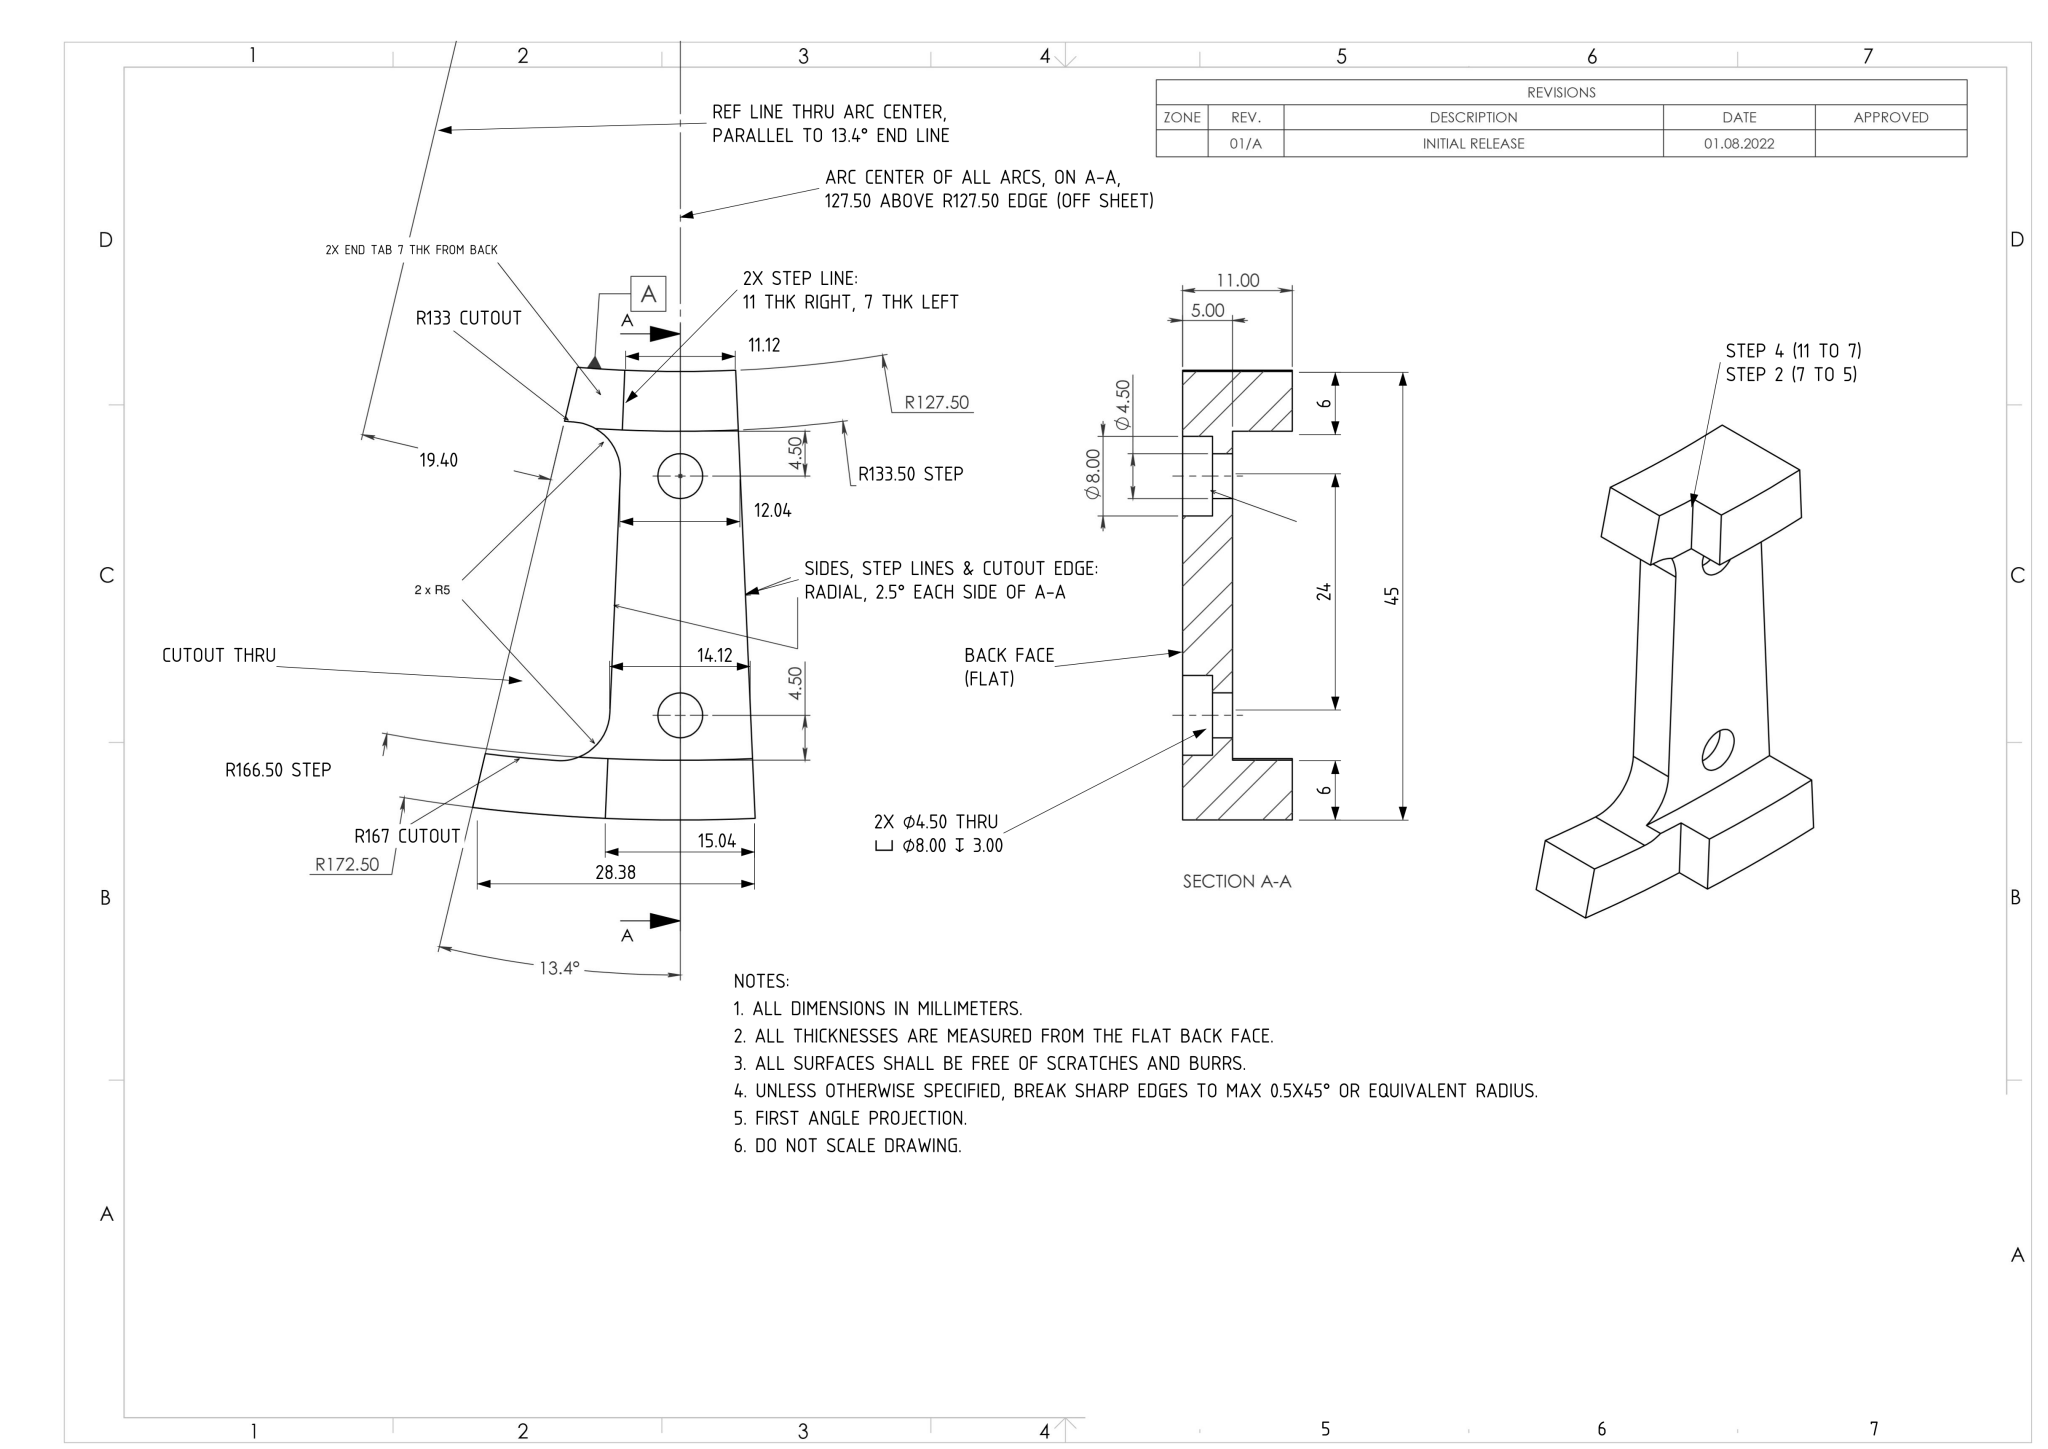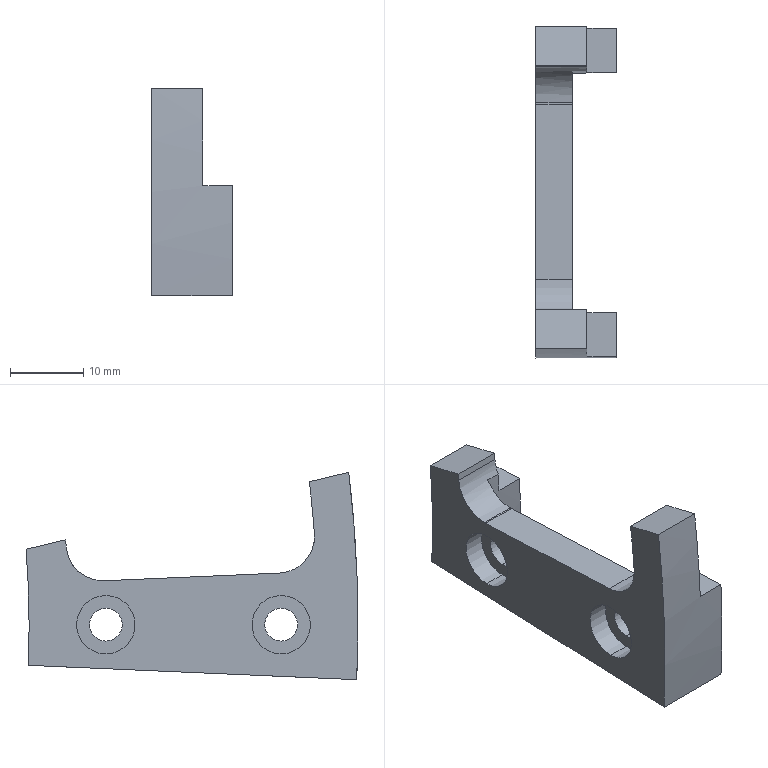Part | NX | mm | 1 solid | 31 faces | box 11 x 45.42 x 28.38 mm | volume 4282 mm3 | cylinder 17 | plane 14 | commonest cylinder face diameters 8 x4 4.5 x4 10 x3 345 x1 255 x1 267 x1 333 x1 266 x1
STEP:
#1=CARTESIAN_POINT('',(-7.131,-137.778,6.016));
#2=VERTEX_POINT('',#1);
#3=CARTESIAN_POINT('',(-7.131,-137.56,6.011));
#4=VERTEX_POINT('',#3);
#5=CARTESIAN_POINT('',(-7.131,-137.56,11.011));
#6=DIRECTION('',(1.,0.,0.));
#7=DIRECTION('',(0.,0.,-1.));
#8=AXIS2_PLACEMENT_3D('',#5,#6,#7);
#9=CIRCLE('',#8,5.);
#10=EDGE_CURVE('',#2,#4,#9,.T.);
#11=ORIENTED_EDGE('',*,*,#10,.T.);
#12=CARTESIAN_POINT('',(-12.131,-137.56,6.011));
#13=VERTEX_POINT('',#12);
#14=CARTESIAN_POINT('',(-5.131,-137.56,6.011));
#15=DIRECTION('',(-1.,0.,0.));
#16=VECTOR('',#15,1000.);
#17=LINE('',#14,#16);
#18=EDGE_CURVE('',#4,#13,#17,.T.);
#19=ORIENTED_EDGE('',*,*,#18,.T.);
#20=CARTESIAN_POINT('',(-12.131,-137.778,6.016));
#21=VERTEX_POINT('',#20);
#22=CARTESIAN_POINT('',(-12.131,-137.56,11.011));
#23=DIRECTION('',(-1.,0.,0.));
#24=DIRECTION('',(0.,0.,1.));
#25=AXIS2_PLACEMENT_3D('',#22,#23,#24);
#26=CIRCLE('',#25,5.);
#27=EDGE_CURVE('',#13,#21,#26,.T.);
#28=ORIENTED_EDGE('',*,*,#27,.T.);
#29=CARTESIAN_POINT('',(-5.131,-137.778,6.016));
#30=DIRECTION('',(1.,0.,0.));
#31=VECTOR('',#30,1000.);
#32=LINE('',#29,#31);
#33=EDGE_CURVE('',#21,#2,#32,.T.);
#34=ORIENTED_EDGE('',*,*,#33,.T.);
#35=EDGE_LOOP('',(#11,#19,#28,#34));
#36=FACE_OUTER_BOUND('',#35,.T.);
#37=CARTESIAN_POINT('',(-5.131,-137.56,11.011));
#38=DIRECTION('',(-1.,0.,0.));
#39=DIRECTION('',(0.,0.,-1.));
#40=AXIS2_PLACEMENT_3D('',#37,#38,#39);
#41=CYLINDRICAL_SURFACE('',#40,5.);
#42=ADVANCED_FACE('',(#36),#41,.F.);
#43=CARTESIAN_POINT('',(-9.131,-138.,-4.));
#44=VERTEX_POINT('',#43);
#45=CARTESIAN_POINT('',(-9.131,-138.,4.));
#46=VERTEX_POINT('',#45);
#47=CARTESIAN_POINT('',(-9.131,-138.,0.));
#48=DIRECTION('',(1.,0.,0.));
#49=DIRECTION('',(0.,0.,-1.));
#50=AXIS2_PLACEMENT_3D('',#47,#48,#49);
#51=CIRCLE('',#50,4.);
#52=EDGE_CURVE('',#44,#46,#51,.T.);
#53=ORIENTED_EDGE('',*,*,#52,.T.);
#54=CARTESIAN_POINT('',(-12.131,-138.,4.));
#55=VERTEX_POINT('',#54);
#56=CARTESIAN_POINT('',(-12.131,-138.,4.));
#57=DIRECTION('',(-1.,0.,0.));
#58=VECTOR('',#57,1000.);
#59=LINE('',#56,#58);
#60=EDGE_CURVE('',#46,#55,#59,.T.);
#61=ORIENTED_EDGE('',*,*,#60,.T.);
#62=CARTESIAN_POINT('',(-12.131,-138.,-4.));
#63=VERTEX_POINT('',#62);
#64=CARTESIAN_POINT('',(-12.131,-138.,0.));
#65=DIRECTION('',(1.,0.,0.));
#66=DIRECTION('',(0.,0.,-1.));
#67=AXIS2_PLACEMENT_3D('',#64,#65,#66);
#68=CIRCLE('',#67,4.);
#69=EDGE_CURVE('',#63,#55,#68,.T.);
#70=ORIENTED_EDGE('',*,*,#69,.F.);
#71=CARTESIAN_POINT('',(-12.131,-138.,-4.));
#72=DIRECTION('',(-1.,0.,0.));
#73=VECTOR('',#72,1000.);
#74=LINE('',#71,#73);
#75=EDGE_CURVE('',#44,#63,#74,.T.);
#76=ORIENTED_EDGE('',*,*,#75,.F.);
#77=EDGE_LOOP('',(#53,#61,#70,#76));
#78=FACE_OUTER_BOUND('',#77,.T.);
#79=CARTESIAN_POINT('',(-12.131,-138.,0.));
#80=DIRECTION('',(-1.,0.,0.));
#81=DIRECTION('',(0.,0.,-1.));
#82=AXIS2_PLACEMENT_3D('',#79,#80,#81);
#83=CYLINDRICAL_SURFACE('',#82,4.);
#84=ADVANCED_FACE('',(#78),#83,.F.);
#85=CARTESIAN_POINT('',(-7.131,-138.,-2.25));
#86=VERTEX_POINT('',#85);
#87=CARTESIAN_POINT('',(-7.131,-138.,2.25));
#88=VERTEX_POINT('',#87);
#89=CARTESIAN_POINT('',(-7.131,-138.,0.));
#90=DIRECTION('',(1.,0.,0.));
#91=DIRECTION('',(0.,0.,-1.));
#92=AXIS2_PLACEMENT_3D('',#89,#90,#91);
#93=CIRCLE('',#92,2.25);
#94=EDGE_CURVE('',#86,#88,#93,.T.);
#95=ORIENTED_EDGE('',*,*,#94,.T.);
#96=CARTESIAN_POINT('',(-9.131,-138.,2.25));
#97=VERTEX_POINT('',#96);
#98=CARTESIAN_POINT('',(-12.131,-138.,2.25));
#99=DIRECTION('',(-1.,0.,0.));
#100=VECTOR('',#99,1000.);
#101=LINE('',#98,#100);
#102=EDGE_CURVE('',#88,#97,#101,.T.);
#103=ORIENTED_EDGE('',*,*,#102,.T.);
#104=CARTESIAN_POINT('',(-9.131,-138.,-2.25));
#105=VERTEX_POINT('',#104);
#106=CARTESIAN_POINT('',(-9.131,-138.,0.));
#107=DIRECTION('',(1.,0.,0.));
#108=DIRECTION('',(0.,0.,-1.));
#109=AXIS2_PLACEMENT_3D('',#106,#107,#108);
#110=CIRCLE('',#109,2.25);
#111=EDGE_CURVE('',#105,#97,#110,.T.);
#112=ORIENTED_EDGE('',*,*,#111,.F.);
#113=CARTESIAN_POINT('',(-12.131,-138.,-2.25));
#114=DIRECTION('',(-1.,0.,0.));
#115=VECTOR('',#114,1000.);
#116=LINE('',#113,#115);
#117=EDGE_CURVE('',#86,#105,#116,.T.);
#118=ORIENTED_EDGE('',*,*,#117,.F.);
#119=EDGE_LOOP('',(#95,#103,#112,#118));
#120=FACE_OUTER_BOUND('',#119,.T.);
#121=CARTESIAN_POINT('',(-12.131,-138.,0.));
#122=DIRECTION('',(-1.,0.,0.));
#123=DIRECTION('',(0.,0.,-1.));
#124=AXIS2_PLACEMENT_3D('',#121,#122,#123);
#125=CYLINDRICAL_SURFACE('',#124,2.25);
#126=ADVANCED_FACE('',(#120),#125,.F.);
#127=CARTESIAN_POINT('',(-9.131,-162.,-4.));
#128=VERTEX_POINT('',#127);
#129=CARTESIAN_POINT('',(-9.131,-162.,4.));
#130=VERTEX_POINT('',#129);
#131=CARTESIAN_POINT('',(-9.131,-162.,0.));
#132=DIRECTION('',(1.,0.,0.));
#133=DIRECTION('',(0.,0.,-1.));
#134=AXIS2_PLACEMENT_3D('',#131,#132,#133);
#135=CIRCLE('',#134,4.);
#136=EDGE_CURVE('',#128,#130,#135,.T.);
#137=ORIENTED_EDGE('',*,*,#136,.T.);
#138=CARTESIAN_POINT('',(-12.131,-162.,4.));
#139=VERTEX_POINT('',#138);
#140=CARTESIAN_POINT('',(-12.131,-162.,4.));
#141=DIRECTION('',(-1.,0.,0.));
#142=VECTOR('',#141,1000.);
#143=LINE('',#140,#142);
#144=EDGE_CURVE('',#130,#139,#143,.T.);
#145=ORIENTED_EDGE('',*,*,#144,.T.);
#146=CARTESIAN_POINT('',(-12.131,-162.,-4.));
#147=VERTEX_POINT('',#146);
#148=CARTESIAN_POINT('',(-12.131,-162.,0.));
#149=DIRECTION('',(1.,0.,0.));
#150=DIRECTION('',(0.,0.,-1.));
#151=AXIS2_PLACEMENT_3D('',#148,#149,#150);
#152=CIRCLE('',#151,4.);
#153=EDGE_CURVE('',#147,#139,#152,.T.);
#154=ORIENTED_EDGE('',*,*,#153,.F.);
#155=CARTESIAN_POINT('',(-12.131,-162.,-4.));
#156=DIRECTION('',(-1.,0.,0.));
#157=VECTOR('',#156,1000.);
#158=LINE('',#155,#157);
#159=EDGE_CURVE('',#128,#147,#158,.T.);
#160=ORIENTED_EDGE('',*,*,#159,.F.);
#161=EDGE_LOOP('',(#137,#145,#154,#160));
#162=FACE_OUTER_BOUND('',#161,.T.);
#163=CARTESIAN_POINT('',(-12.131,-162.,0.));
#164=DIRECTION('',(-1.,0.,0.));
#165=DIRECTION('',(0.,0.,-1.));
#166=AXIS2_PLACEMENT_3D('',#163,#164,#165);
#167=CYLINDRICAL_SURFACE('',#166,4.);
#168=ADVANCED_FACE('',(#162),#167,.F.);
#169=CARTESIAN_POINT('',(-7.131,-162.,-2.25));
#170=VERTEX_POINT('',#169);
#171=CARTESIAN_POINT('',(-7.131,-162.,2.25));
#172=VERTEX_POINT('',#171);
#173=CARTESIAN_POINT('',(-7.131,-162.,0.));
#174=DIRECTION('',(1.,0.,0.));
#175=DIRECTION('',(0.,0.,-1.));
#176=AXIS2_PLACEMENT_3D('',#173,#174,#175);
#177=CIRCLE('',#176,2.25);
#178=EDGE_CURVE('',#170,#172,#177,.T.);
#179=ORIENTED_EDGE('',*,*,#178,.T.);
#180=CARTESIAN_POINT('',(-9.131,-162.,2.25));
#181=VERTEX_POINT('',#180);
#182=CARTESIAN_POINT('',(-12.131,-162.,2.25));
#183=DIRECTION('',(-1.,0.,0.));
#184=VECTOR('',#183,1000.);
#185=LINE('',#182,#184);
#186=EDGE_CURVE('',#172,#181,#185,.T.);
#187=ORIENTED_EDGE('',*,*,#186,.T.);
#188=CARTESIAN_POINT('',(-9.131,-162.,-2.25));
#189=VERTEX_POINT('',#188);
#190=CARTESIAN_POINT('',(-9.131,-162.,0.));
#191=DIRECTION('',(1.,0.,0.));
#192=DIRECTION('',(0.,0.,-1.));
#193=AXIS2_PLACEMENT_3D('',#190,#191,#192);
#194=CIRCLE('',#193,2.25);
#195=EDGE_CURVE('',#189,#181,#194,.T.);
#196=ORIENTED_EDGE('',*,*,#195,.F.);
#197=CARTESIAN_POINT('',(-12.131,-162.,-2.25));
#198=DIRECTION('',(-1.,0.,0.));
#199=VECTOR('',#198,1000.);
#200=LINE('',#197,#199);
#201=EDGE_CURVE('',#170,#189,#200,.T.);
#202=ORIENTED_EDGE('',*,*,#201,.F.);
#203=EDGE_LOOP('',(#179,#187,#196,#202));
#204=FACE_OUTER_BOUND('',#203,.T.);
#205=CARTESIAN_POINT('',(-12.131,-162.,0.));
#206=DIRECTION('',(-1.,0.,0.));
#207=DIRECTION('',(0.,0.,-1.));
#208=AXIS2_PLACEMENT_3D('',#205,#206,#207);
#209=CYLINDRICAL_SURFACE('',#208,2.25);
#210=ADVANCED_FACE('',(#204),#209,.F.);
#211=CARTESIAN_POINT('',(-7.131,-161.769,7.063));
#212=VERTEX_POINT('',#211);
#213=CARTESIAN_POINT('',(-7.131,-133.373,5.823));
#214=DIRECTION('',(-0.,0.999,-0.04362));
#215=VECTOR('',#214,1000.);
#216=LINE('',#213,#215);
#217=EDGE_CURVE('',#212,#2,#216,.T.);
#218=ORIENTED_EDGE('',*,*,#217,.T.);
#219=ORIENTED_EDGE('',*,*,#33,.F.);
#220=CARTESIAN_POINT('',(-12.131,-161.769,7.063));
#221=VERTEX_POINT('',#220);
#222=CARTESIAN_POINT('',(-12.131,-133.373,5.823));
#223=DIRECTION('',(0.,-0.999,0.04362));
#224=VECTOR('',#223,1000.);
#225=LINE('',#222,#224);
#226=EDGE_CURVE('',#21,#221,#225,.T.);
#227=ORIENTED_EDGE('',*,*,#226,.T.);
#228=CARTESIAN_POINT('',(-12.131,-161.769,7.063));
#229=DIRECTION('',(-1.,0.,0.));
#230=VECTOR('',#229,1000.);
#231=LINE('',#228,#230);
#232=EDGE_CURVE('',#212,#221,#231,.T.);
#233=ORIENTED_EDGE('',*,*,#232,.F.);
#234=EDGE_LOOP('',(#218,#219,#227,#233));
#235=FACE_OUTER_BOUND('',#234,.T.);
#236=CARTESIAN_POINT('',(0.,0.,0.));
#237=DIRECTION('',(0.,0.04362,0.999));
#238=DIRECTION('',(-1.,0.,0.));
#239=AXIS2_PLACEMENT_3D('',#236,#237,#238);
#240=PLANE('',#239);
#241=ADVANCED_FACE('',(#235),#240,.T.);
#242=CARTESIAN_POINT('',(-5.131,-172.336,7.524));
#243=VERTEX_POINT('',#242);
#244=CARTESIAN_POINT('',(-5.131,-166.342,7.263));
#245=VERTEX_POINT('',#244);
#246=CARTESIAN_POINT('',(-5.131,-166.841,7.284));
#247=DIRECTION('',(0.,0.999,-0.04362));
#248=VECTOR('',#247,1000.);
#249=LINE('',#246,#248);
#250=EDGE_CURVE('',#243,#245,#249,.T.);
#251=ORIENTED_EDGE('',*,*,#250,.F.);
#252=CARTESIAN_POINT('',(-1.131,-172.336,7.524));
#253=VERTEX_POINT('',#252);
#254=CARTESIAN_POINT('',(-12.131,-172.336,7.524));
#255=DIRECTION('',(1.,0.,0.));
#256=VECTOR('',#255,1000.);
#257=LINE('',#254,#256);
#258=EDGE_CURVE('',#243,#253,#257,.T.);
#259=ORIENTED_EDGE('',*,*,#258,.T.);
#260=CARTESIAN_POINT('',(-1.131,-166.342,7.263));
#261=VERTEX_POINT('',#260);
#262=CARTESIAN_POINT('',(-1.131,0.,0.));
#263=DIRECTION('',(0.,0.999,-0.04362));
#264=VECTOR('',#263,1000.);
#265=LINE('',#262,#264);
#266=EDGE_CURVE('',#253,#261,#265,.T.);
#267=ORIENTED_EDGE('',*,*,#266,.T.);
#268=CARTESIAN_POINT('',(-1.131,-166.342,7.263));
#269=DIRECTION('',(-1.,0.,0.));
#270=VECTOR('',#269,1000.);
#271=LINE('',#268,#270);
#272=EDGE_CURVE('',#261,#245,#271,.T.);
#273=ORIENTED_EDGE('',*,*,#272,.T.);
#274=EDGE_LOOP('',(#251,#259,#267,#273));
#275=FACE_OUTER_BOUND('',#274,.T.);
#276=CARTESIAN_POINT('',(0.,0.,0.));
#277=DIRECTION('',(0.,0.04362,0.999));
#278=DIRECTION('',(-1.,0.,0.));
#279=AXIS2_PLACEMENT_3D('',#276,#277,#278);
#280=PLANE('',#279);
#281=ADVANCED_FACE('',(#275),#280,.T.);
#282=CARTESIAN_POINT('',(-12.131,-127.379,-5.561));
#283=VERTEX_POINT('',#282);
#284=CARTESIAN_POINT('',(-12.131,-127.081,10.332));
#285=VERTEX_POINT('',#284);
#286=CARTESIAN_POINT('',(-12.131,0.,0.));
#287=DIRECTION('',(-1.,0.,0.));
#288=DIRECTION('',(0.,0.,1.));
#289=AXIS2_PLACEMENT_3D('',#286,#287,#288);
#290=CIRCLE('',#289,127.5);
#291=EDGE_CURVE('',#283,#285,#290,.T.);
#292=ORIENTED_EDGE('',*,*,#291,.F.);
#293=CARTESIAN_POINT('',(-12.131,-172.336,-7.524));
#294=VERTEX_POINT('',#293);
#295=CARTESIAN_POINT('',(-12.131,-133.373,-5.823));
#296=DIRECTION('',(0.,-0.999,-0.04362));
#297=VECTOR('',#296,1000.);
#298=LINE('',#295,#297);
#299=EDGE_CURVE('',#283,#294,#298,.T.);
#300=ORIENTED_EDGE('',*,*,#299,.T.);
#301=CARTESIAN_POINT('',(-12.131,-171.235,20.851));
#302=VERTEX_POINT('',#301);
#303=CARTESIAN_POINT('',(-12.131,0.,0.));
#304=DIRECTION('',(-1.,0.,0.));
#305=DIRECTION('',(0.,0.,1.));
#306=AXIS2_PLACEMENT_3D('',#303,#304,#305);
#307=CIRCLE('',#306,172.5);
#308=EDGE_CURVE('',#294,#302,#307,.T.);
#309=ORIENTED_EDGE('',*,*,#308,.T.);
#310=CARTESIAN_POINT('',(-12.131,-165.85,19.568));
#311=VERTEX_POINT('',#310);
#312=CARTESIAN_POINT('',(-12.131,-165.85,19.568));
#313=DIRECTION('',(0.,-0.9728,0.2317));
#314=VECTOR('',#313,1000.);
#315=LINE('',#312,#314);
#316=EDGE_CURVE('',#311,#302,#315,.T.);
#317=ORIENTED_EDGE('',*,*,#316,.F.);
#318=CARTESIAN_POINT('',(-12.131,-166.537,12.43));
#319=VERTEX_POINT('',#318);
#320=CARTESIAN_POINT('',(-12.131,0.,0.));
#321=DIRECTION('',(-1.,0.,0.));
#322=DIRECTION('',(0.,0.,-1.));
#323=AXIS2_PLACEMENT_3D('',#320,#321,#322);
#324=CIRCLE('',#323,167.);
#325=EDGE_CURVE('',#319,#311,#324,.T.);
#326=ORIENTED_EDGE('',*,*,#325,.F.);
#327=CARTESIAN_POINT('',(-12.131,-161.551,12.058));
#328=DIRECTION('',(-1.,0.,0.));
#329=DIRECTION('',(0.,0.,1.));
#330=AXIS2_PLACEMENT_3D('',#327,#328,#329);
#331=CIRCLE('',#330,5.);
#332=EDGE_CURVE('',#221,#319,#331,.T.);
#333=ORIENTED_EDGE('',*,*,#332,.F.);
#334=ORIENTED_EDGE('',*,*,#226,.F.);
#335=ORIENTED_EDGE('',*,*,#27,.F.);
#336=CARTESIAN_POINT('',(-12.131,-132.576,10.612));
#337=VERTEX_POINT('',#336);
#338=CARTESIAN_POINT('',(-12.131,-137.56,11.011));
#339=DIRECTION('',(-1.,0.,0.));
#340=DIRECTION('',(0.,0.,1.));
#341=AXIS2_PLACEMENT_3D('',#338,#339,#340);
#342=CIRCLE('',#341,5.);
#343=EDGE_CURVE('',#337,#13,#342,.T.);
#344=ORIENTED_EDGE('',*,*,#343,.F.);
#345=CARTESIAN_POINT('',(-12.131,-132.491,11.621));
#346=VERTEX_POINT('',#345);
#347=CARTESIAN_POINT('',(-12.131,0.,0.));
#348=DIRECTION('',(1.,0.,0.));
#349=DIRECTION('',(0.,0.,-1.));
#350=AXIS2_PLACEMENT_3D('',#347,#348,#349);
#351=CIRCLE('',#350,133.);
#352=EDGE_CURVE('',#346,#337,#351,.T.);
#353=ORIENTED_EDGE('',*,*,#352,.F.);
#354=CARTESIAN_POINT('',(-12.131,-127.081,10.332));
#355=DIRECTION('',(0.,-0.9728,0.2317));
#356=VECTOR('',#355,1000.);
#357=LINE('',#354,#356);
#358=EDGE_CURVE('',#285,#346,#357,.T.);
#359=ORIENTED_EDGE('',*,*,#358,.F.);
#360=EDGE_LOOP('',(#292,#300,#309,#317,#326,#333,#334,#335,#344,#353,#359));
#361=FACE_OUTER_BOUND('',#360,.T.);
#362=ORIENTED_EDGE('',*,*,#153,.T.);
#363=CARTESIAN_POINT('',(-12.131,-162.,0.));
#364=DIRECTION('',(1.,0.,0.));
#365=DIRECTION('',(0.,0.,-1.));
#366=AXIS2_PLACEMENT_3D('',#363,#364,#365);
#367=CIRCLE('',#366,4.);
#368=EDGE_CURVE('',#139,#147,#367,.T.);
#369=ORIENTED_EDGE('',*,*,#368,.T.);
#370=EDGE_LOOP('',(#362,#369));
#371=FACE_BOUND('',#370,.T.);
#372=ORIENTED_EDGE('',*,*,#69,.T.);
#373=CARTESIAN_POINT('',(-12.131,-138.,0.));
#374=DIRECTION('',(1.,0.,0.));
#375=DIRECTION('',(0.,0.,-1.));
#376=AXIS2_PLACEMENT_3D('',#373,#374,#375);
#377=CIRCLE('',#376,4.);
#378=EDGE_CURVE('',#55,#63,#377,.T.);
#379=ORIENTED_EDGE('',*,*,#378,.T.);
#380=EDGE_LOOP('',(#372,#379));
#381=FACE_BOUND('',#380,.T.);
#382=CARTESIAN_POINT('',(-12.131,-133.373,-5.823));
#383=DIRECTION('',(1.,0.,0.));
#384=DIRECTION('',(0.,0.,1.));
#385=AXIS2_PLACEMENT_3D('',#382,#383,#384);
#386=PLANE('',#385);
#387=ADVANCED_FACE('',(#361,#371,#381),#386,.F.);
#388=ORIENTED_EDGE('',*,*,#94,.F.);
#389=CARTESIAN_POINT('',(-7.131,-138.,0.));
#390=DIRECTION('',(1.,0.,0.));
#391=DIRECTION('',(0.,0.,-1.));
#392=AXIS2_PLACEMENT_3D('',#389,#390,#391);
#393=CIRCLE('',#392,2.25);
#394=EDGE_CURVE('',#88,#86,#393,.T.);
#395=ORIENTED_EDGE('',*,*,#394,.F.);
#396=EDGE_LOOP('',(#388,#395));
#397=FACE_BOUND('',#396,.T.);
#398=ORIENTED_EDGE('',*,*,#178,.F.);
#399=CARTESIAN_POINT('',(-7.131,-162.,0.));
#400=DIRECTION('',(1.,0.,0.));
#401=DIRECTION('',(0.,0.,-1.));
#402=AXIS2_PLACEMENT_3D('',#399,#400,#401);
#403=CIRCLE('',#402,2.25);
#404=EDGE_CURVE('',#172,#170,#403,.T.);
#405=ORIENTED_EDGE('',*,*,#404,.F.);
#406=EDGE_LOOP('',(#398,#405));
#407=FACE_BOUND('',#406,.T.);
#408=CARTESIAN_POINT('',(-7.131,-166.342,-7.263));
#409=VERTEX_POINT('',#408);
#410=CARTESIAN_POINT('',(-7.131,-133.373,-5.823));
#411=VERTEX_POINT('',#410);
#412=CARTESIAN_POINT('',(-7.131,-133.373,-5.823));
#413=DIRECTION('',(-0.,0.999,0.04362));
#414=VECTOR('',#413,1000.);
#415=LINE('',#412,#414);
#416=EDGE_CURVE('',#409,#411,#415,.T.);
#417=ORIENTED_EDGE('',*,*,#416,.T.);
#418=CARTESIAN_POINT('',(-7.131,-133.228,8.514));
#419=VERTEX_POINT('',#418);
#420=CARTESIAN_POINT('',(-7.131,0.,0.));
#421=DIRECTION('',(-1.,0.,0.));
#422=DIRECTION('',(0.,0.,1.));
#423=AXIS2_PLACEMENT_3D('',#420,#421,#422);
#424=CIRCLE('',#423,133.5);
#425=EDGE_CURVE('',#411,#419,#424,.T.);
#426=ORIENTED_EDGE('',*,*,#425,.T.);
#427=CARTESIAN_POINT('',(-7.131,-137.56,11.011));
#428=DIRECTION('',(1.,0.,0.));
#429=DIRECTION('',(0.,0.,-1.));
#430=AXIS2_PLACEMENT_3D('',#427,#428,#429);
#431=CIRCLE('',#430,5.);
#432=EDGE_CURVE('',#4,#419,#431,.T.);
#433=ORIENTED_EDGE('',*,*,#432,.F.);
#434=ORIENTED_EDGE('',*,*,#10,.F.);
#435=ORIENTED_EDGE('',*,*,#217,.F.);
#436=CARTESIAN_POINT('',(-7.131,-166.188,10.189));
#437=VERTEX_POINT('',#436);
#438=CARTESIAN_POINT('',(-7.131,-161.551,12.058));
#439=DIRECTION('',(1.,0.,0.));
#440=DIRECTION('',(0.,0.,-1.));
#441=AXIS2_PLACEMENT_3D('',#438,#439,#440);
#442=CIRCLE('',#441,5.);
#443=EDGE_CURVE('',#437,#212,#442,.T.);
#444=ORIENTED_EDGE('',*,*,#443,.F.);
#445=CARTESIAN_POINT('',(-7.131,0.,0.));
#446=DIRECTION('',(-1.,0.,0.));
#447=DIRECTION('',(0.,0.,1.));
#448=AXIS2_PLACEMENT_3D('',#445,#446,#447);
#449=CIRCLE('',#448,166.5);
#450=EDGE_CURVE('',#409,#437,#449,.T.);
#451=ORIENTED_EDGE('',*,*,#450,.F.);
#452=EDGE_LOOP('',(#417,#426,#433,#434,#435,#444,#451));
#453=FACE_OUTER_BOUND('',#452,.T.);
#454=CARTESIAN_POINT('',(-7.131,-133.373,-5.823));
#455=DIRECTION('',(-1.,0.,0.));
#456=DIRECTION('',(0.,0.,-1.));
#457=AXIS2_PLACEMENT_3D('',#454,#455,#456);
#458=PLANE('',#457);
#459=ADVANCED_FACE('',(#397,#407,#453),#458,.F.);
#460=ORIENTED_EDGE('',*,*,#308,.F.);
#461=CARTESIAN_POINT('',(-1.131,-172.336,-7.524));
#462=VERTEX_POINT('',#461);
#463=CARTESIAN_POINT('',(0.,-172.336,-7.524));
#464=DIRECTION('',(1.,0.,0.));
#465=VECTOR('',#464,1000.);
#466=LINE('',#463,#465);
#467=EDGE_CURVE('',#294,#462,#466,.T.);
#468=ORIENTED_EDGE('',*,*,#467,.T.);
#469=CARTESIAN_POINT('',(-1.131,0.,0.));
#470=DIRECTION('',(-1.,0.,0.));
#471=DIRECTION('',(0.,0.,1.));
#472=AXIS2_PLACEMENT_3D('',#469,#470,#471);
#473=CIRCLE('',#472,172.5);
#474=EDGE_CURVE('',#462,#253,#473,.T.);
#475=ORIENTED_EDGE('',*,*,#474,.T.);
#476=ORIENTED_EDGE('',*,*,#258,.F.);
#477=CARTESIAN_POINT('',(-5.131,-171.235,20.851));
#478=VERTEX_POINT('',#477);
#479=CARTESIAN_POINT('',(-5.131,0.,0.));
#480=DIRECTION('',(1.,0.,0.));
#481=DIRECTION('',(0.,0.,-1.));
#482=AXIS2_PLACEMENT_3D('',#479,#480,#481);
#483=CIRCLE('',#482,172.5);
#484=EDGE_CURVE('',#478,#243,#483,.T.);
#485=ORIENTED_EDGE('',*,*,#484,.F.);
#486=CARTESIAN_POINT('',(-5.131,-171.235,20.851));
#487=DIRECTION('',(-1.,0.,0.));
#488=VECTOR('',#487,1000.);
#489=LINE('',#486,#488);
#490=EDGE_CURVE('',#478,#302,#489,.T.);
#491=ORIENTED_EDGE('',*,*,#490,.T.);
#492=EDGE_LOOP('',(#460,#468,#475,#476,#485,#491));
#493=FACE_OUTER_BOUND('',#492,.T.);
#494=CARTESIAN_POINT('',(0.,0.,0.));
#495=DIRECTION('',(1.,0.,0.));
#496=DIRECTION('',(0.,0.,1.));
#497=AXIS2_PLACEMENT_3D('',#494,#495,#496);
#498=CYLINDRICAL_SURFACE('',#497,172.5);
#499=ADVANCED_FACE('',(#493),#498,.T.);
#500=CARTESIAN_POINT('',(-1.131,-127.379,-5.561));
#501=VERTEX_POINT('',#500);
#502=CARTESIAN_POINT('',(0.,-127.379,-5.561));
#503=DIRECTION('',(-1.,0.,0.));
#504=VECTOR('',#503,1000.);
#505=LINE('',#502,#504);
#506=EDGE_CURVE('',#501,#283,#505,.T.);
#507=ORIENTED_EDGE('',*,*,#506,.T.);
#508=ORIENTED_EDGE('',*,*,#291,.T.);
#509=CARTESIAN_POINT('',(-5.131,-127.081,10.332));
#510=VERTEX_POINT('',#509);
#511=CARTESIAN_POINT('',(-5.131,-127.081,10.332));
#512=DIRECTION('',(-1.,0.,0.));
#513=VECTOR('',#512,1000.);
#514=LINE('',#511,#513);
#515=EDGE_CURVE('',#510,#285,#514,.T.);
#516=ORIENTED_EDGE('',*,*,#515,.F.);
#517=CARTESIAN_POINT('',(-5.131,-127.379,5.561));
#518=VERTEX_POINT('',#517);
#519=CARTESIAN_POINT('',(-5.131,0.,0.));
#520=DIRECTION('',(-1.,0.,0.));
#521=DIRECTION('',(0.,0.,-1.));
#522=AXIS2_PLACEMENT_3D('',#519,#520,#521);
#523=CIRCLE('',#522,127.5);
#524=EDGE_CURVE('',#518,#510,#523,.T.);
#525=ORIENTED_EDGE('',*,*,#524,.F.);
#526=CARTESIAN_POINT('',(-1.131,-127.379,5.561));
#527=VERTEX_POINT('',#526);
#528=CARTESIAN_POINT('',(0.,-127.379,5.561));
#529=DIRECTION('',(-1.,0.,0.));
#530=VECTOR('',#529,1000.);
#531=LINE('',#528,#530);
#532=EDGE_CURVE('',#527,#518,#531,.T.);
#533=ORIENTED_EDGE('',*,*,#532,.F.);
#534=CARTESIAN_POINT('',(-1.131,0.,0.));
#535=DIRECTION('',(1.,0.,0.));
#536=DIRECTION('',(0.,0.,1.));
#537=AXIS2_PLACEMENT_3D('',#534,#535,#536);
#538=CIRCLE('',#537,127.5);
#539=EDGE_CURVE('',#527,#501,#538,.T.);
#540=ORIENTED_EDGE('',*,*,#539,.T.);
#541=EDGE_LOOP('',(#507,#508,#516,#525,#533,#540));
#542=FACE_OUTER_BOUND('',#541,.T.);
#543=CARTESIAN_POINT('',(0.,0.,0.));
#544=DIRECTION('',(1.,0.,0.));
#545=DIRECTION('',(0.,0.,1.));
#546=AXIS2_PLACEMENT_3D('',#543,#544,#545);
#547=CYLINDRICAL_SURFACE('',#546,127.5);
#548=ADVANCED_FACE('',(#542),#547,.F.);
#549=ORIENTED_EDGE('',*,*,#467,.F.);
#550=ORIENTED_EDGE('',*,*,#299,.F.);
#551=ORIENTED_EDGE('',*,*,#506,.F.);
#552=CARTESIAN_POINT('',(-1.131,-133.373,-5.823));
#553=VERTEX_POINT('',#552);
#554=CARTESIAN_POINT('',(-1.131,0.,0.));
#555=DIRECTION('',(0.,-0.999,-0.04362));
#556=VECTOR('',#555,1000.);
#557=LINE('',#554,#556);
#558=EDGE_CURVE('',#501,#553,#557,.T.);
#559=ORIENTED_EDGE('',*,*,#558,.T.);
#560=CARTESIAN_POINT('',(-1.131,-133.373,-5.823));
#561=DIRECTION('',(-1.,0.,0.));
#562=VECTOR('',#561,1000.);
#563=LINE('',#560,#562);
#564=EDGE_CURVE('',#553,#411,#563,.T.);
#565=ORIENTED_EDGE('',*,*,#564,.T.);
#566=ORIENTED_EDGE('',*,*,#416,.F.);
#567=CARTESIAN_POINT('',(-1.131,-166.342,-7.263));
#568=VERTEX_POINT('',#567);
#569=CARTESIAN_POINT('',(-1.131,-166.342,-7.263));
#570=DIRECTION('',(-1.,0.,0.));
#571=VECTOR('',#570,1000.);
#572=LINE('',#569,#571);
#573=EDGE_CURVE('',#568,#409,#572,.T.);
#574=ORIENTED_EDGE('',*,*,#573,.F.);
#575=CARTESIAN_POINT('',(-1.131,0.,0.));
#576=DIRECTION('',(0.,-0.999,-0.04362));
#577=VECTOR('',#576,1000.);
#578=LINE('',#575,#577);
#579=EDGE_CURVE('',#568,#462,#578,.T.);
#580=ORIENTED_EDGE('',*,*,#579,.T.);
#581=EDGE_LOOP('',(#549,#550,#551,#559,#565,#566,#574,#580));
#582=FACE_OUTER_BOUND('',#581,.T.);
#583=CARTESIAN_POINT('',(0.,0.,0.));
#584=DIRECTION('',(0.,-0.04362,0.999));
#585=DIRECTION('',(-1.,0.,0.));
#586=AXIS2_PLACEMENT_3D('',#583,#584,#585);
#587=PLANE('',#586);
#588=ADVANCED_FACE('',(#582),#587,.F.);
#589=CARTESIAN_POINT('',(-1.131,-133.373,5.823));
#590=VERTEX_POINT('',#589);
#591=CARTESIAN_POINT('',(-5.131,-133.373,5.823));
#592=VERTEX_POINT('',#591);
#593=CARTESIAN_POINT('',(-1.131,-133.373,5.823));
#594=DIRECTION('',(-1.,0.,0.));
#595=VECTOR('',#594,1000.);
#596=LINE('',#593,#595);
#597=EDGE_CURVE('',#590,#592,#596,.T.);
#598=ORIENTED_EDGE('',*,*,#597,.F.);
#599=CARTESIAN_POINT('',(-1.131,0.,0.));
#600=DIRECTION('',(0.,0.999,-0.04362));
#601=VECTOR('',#600,1000.);
#602=LINE('',#599,#601);
#603=EDGE_CURVE('',#590,#527,#602,.T.);
#604=ORIENTED_EDGE('',*,*,#603,.T.);
#605=ORIENTED_EDGE('',*,*,#532,.T.);
#606=CARTESIAN_POINT('',(-5.131,-127.379,5.561));
#607=DIRECTION('',(0.,0.999,-0.04362));
#608=VECTOR('',#607,1000.);
#609=LINE('',#606,#608);
#610=EDGE_CURVE('',#592,#518,#609,.T.);
#611=ORIENTED_EDGE('',*,*,#610,.F.);
#612=EDGE_LOOP('',(#598,#604,#605,#611));
#613=FACE_OUTER_BOUND('',#612,.T.);
#614=CARTESIAN_POINT('',(0.,0.,0.));
#615=DIRECTION('',(0.,0.04362,0.999));
#616=DIRECTION('',(-1.,0.,0.));
#617=AXIS2_PLACEMENT_3D('',#614,#615,#616);
#618=PLANE('',#617);
#619=ADVANCED_FACE('',(#613),#618,.T.);
#620=ORIENTED_EDGE('',*,*,#425,.F.);
#621=ORIENTED_EDGE('',*,*,#564,.F.);
#622=CARTESIAN_POINT('',(-1.131,0.,0.));
#623=DIRECTION('',(-1.,0.,0.));
#624=DIRECTION('',(0.,0.,1.));
#625=AXIS2_PLACEMENT_3D('',#622,#623,#624);
#626=CIRCLE('',#625,133.5);
#627=EDGE_CURVE('',#553,#590,#626,.T.);
#628=ORIENTED_EDGE('',*,*,#627,.T.);
#629=ORIENTED_EDGE('',*,*,#597,.T.);
#630=CARTESIAN_POINT('',(-5.131,-133.228,8.514));
#631=VERTEX_POINT('',#630);
#632=CARTESIAN_POINT('',(-5.131,0.,0.));
#633=DIRECTION('',(-1.,0.,0.));
#634=DIRECTION('',(0.,0.,-1.));
#635=AXIS2_PLACEMENT_3D('',#632,#633,#634);
#636=CIRCLE('',#635,133.5);
#637=EDGE_CURVE('',#592,#631,#636,.T.);
#638=ORIENTED_EDGE('',*,*,#637,.T.);
#639=CARTESIAN_POINT('',(-5.131,-133.228,8.514));
#640=DIRECTION('',(1.,0.,0.));
#641=VECTOR('',#640,1000.);
#642=LINE('',#639,#641);
#643=EDGE_CURVE('',#419,#631,#642,.T.);
#644=ORIENTED_EDGE('',*,*,#643,.F.);
#645=EDGE_LOOP('',(#620,#621,#628,#629,#638,#644));
#646=FACE_OUTER_BOUND('',#645,.T.);
#647=CARTESIAN_POINT('',(-1.131,0.,0.));
#648=DIRECTION('',(-1.,0.,0.));
#649=DIRECTION('',(0.,0.,-1.));
#650=AXIS2_PLACEMENT_3D('',#647,#648,#649);
#651=CYLINDRICAL_SURFACE('',#650,133.5);
#652=ADVANCED_FACE('',(#646),#651,.T.);
#653=ORIENTED_EDGE('',*,*,#558,.F.);
#654=ORIENTED_EDGE('',*,*,#539,.F.);
#655=ORIENTED_EDGE('',*,*,#603,.F.);
#656=ORIENTED_EDGE('',*,*,#627,.F.);
#657=EDGE_LOOP('',(#653,#654,#655,#656));
#658=FACE_OUTER_BOUND('',#657,.T.);
#659=CARTESIAN_POINT('',(-1.131,0.,0.));
#660=DIRECTION('',(1.,0.,0.));
#661=DIRECTION('',(0.,0.,1.));
#662=AXIS2_PLACEMENT_3D('',#659,#660,#661);
#663=PLANE('',#662);
#664=ADVANCED_FACE('',(#658),#663,.T.);
#665=ORIENTED_EDGE('',*,*,#450,.T.);
#666=CARTESIAN_POINT('',(-5.131,-166.188,10.189));
#667=VERTEX_POINT('',#666);
#668=CARTESIAN_POINT('',(-1.131,-166.188,10.189));
#669=DIRECTION('',(-1.,0.,0.));
#670=VECTOR('',#669,1000.);
#671=LINE('',#668,#670);
#672=EDGE_CURVE('',#667,#437,#671,.T.);
#673=ORIENTED_EDGE('',*,*,#672,.F.);
#674=CARTESIAN_POINT('',(-5.131,0.,0.));
#675=DIRECTION('',(-1.,0.,0.));
#676=DIRECTION('',(0.,0.,-1.));
#677=AXIS2_PLACEMENT_3D('',#674,#675,#676);
#678=CIRCLE('',#677,166.5);
#679=EDGE_CURVE('',#245,#667,#678,.T.);
#680=ORIENTED_EDGE('',*,*,#679,.F.);
#681=ORIENTED_EDGE('',*,*,#272,.F.);
#682=CARTESIAN_POINT('',(-1.131,0.,0.));
#683=DIRECTION('',(-1.,0.,0.));
#684=DIRECTION('',(0.,0.,1.));
#685=AXIS2_PLACEMENT_3D('',#682,#683,#684);
#686=CIRCLE('',#685,166.5);
#687=EDGE_CURVE('',#568,#261,#686,.T.);
#688=ORIENTED_EDGE('',*,*,#687,.F.);
#689=ORIENTED_EDGE('',*,*,#573,.T.);
#690=EDGE_LOOP('',(#665,#673,#680,#681,#688,#689));
#691=FACE_OUTER_BOUND('',#690,.T.);
#692=CARTESIAN_POINT('',(-1.131,0.,0.));
#693=DIRECTION('',(-1.,0.,0.));
#694=DIRECTION('',(0.,0.,-1.));
#695=AXIS2_PLACEMENT_3D('',#692,#693,#694);
#696=CYLINDRICAL_SURFACE('',#695,166.5);
#697=ADVANCED_FACE('',(#691),#696,.F.);
#698=ORIENTED_EDGE('',*,*,#687,.T.);
#699=ORIENTED_EDGE('',*,*,#266,.F.);
#700=ORIENTED_EDGE('',*,*,#474,.F.);
#701=ORIENTED_EDGE('',*,*,#579,.F.);
#702=EDGE_LOOP('',(#698,#699,#700,#701));
#703=FACE_OUTER_BOUND('',#702,.T.);
#704=CARTESIAN_POINT('',(-1.131,0.,0.));
#705=DIRECTION('',(1.,0.,0.));
#706=DIRECTION('',(0.,0.,1.));
#707=AXIS2_PLACEMENT_3D('',#704,#705,#706);
#708=PLANE('',#707);
#709=ADVANCED_FACE('',(#703),#708,.T.);
#710=CARTESIAN_POINT('',(-5.131,-132.491,11.621));
#711=VERTEX_POINT('',#710);
#712=CARTESIAN_POINT('',(-5.131,-132.576,10.612));
#713=VERTEX_POINT('',#712);
#714=CARTESIAN_POINT('',(-5.131,0.,0.));
#715=DIRECTION('',(1.,0.,0.));
#716=DIRECTION('',(0.,0.,-1.));
#717=AXIS2_PLACEMENT_3D('',#714,#715,#716);
#718=CIRCLE('',#717,133.);
#719=EDGE_CURVE('',#711,#713,#718,.T.);
#720=ORIENTED_EDGE('',*,*,#719,.F.);
#721=CARTESIAN_POINT('',(-5.131,-132.491,11.621));
#722=DIRECTION('',(-1.,0.,0.));
#723=VECTOR('',#722,1000.);
#724=LINE('',#721,#723);
#725=EDGE_CURVE('',#711,#346,#724,.T.);
#726=ORIENTED_EDGE('',*,*,#725,.T.);
#727=ORIENTED_EDGE('',*,*,#352,.T.);
#728=CARTESIAN_POINT('',(-5.131,-132.576,10.612));
#729=DIRECTION('',(-1.,0.,0.));
#730=VECTOR('',#729,1000.);
#731=LINE('',#728,#730);
#732=EDGE_CURVE('',#713,#337,#731,.T.);
#733=ORIENTED_EDGE('',*,*,#732,.F.);
#734=EDGE_LOOP('',(#720,#726,#727,#733));
#735=FACE_OUTER_BOUND('',#734,.T.);
#736=CARTESIAN_POINT('',(-5.131,0.,0.));
#737=DIRECTION('',(-1.,0.,0.));
#738=DIRECTION('',(0.,0.,-1.));
#739=AXIS2_PLACEMENT_3D('',#736,#737,#738);
#740=CYLINDRICAL_SURFACE('',#739,133.);
#741=ADVANCED_FACE('',(#735),#740,.T.);
#742=ORIENTED_EDGE('',*,*,#358,.T.);
#743=ORIENTED_EDGE('',*,*,#725,.F.);
#744=CARTESIAN_POINT('',(-5.131,-127.081,10.332));
#745=DIRECTION('',(0.,-0.9728,0.2317));
#746=VECTOR('',#745,1000.);
#747=LINE('',#744,#746);
#748=EDGE_CURVE('',#510,#711,#747,.T.);
#749=ORIENTED_EDGE('',*,*,#748,.F.);
#750=ORIENTED_EDGE('',*,*,#515,.T.);
#751=EDGE_LOOP('',(#742,#743,#749,#750));
#752=FACE_OUTER_BOUND('',#751,.T.);
#753=CARTESIAN_POINT('',(-5.131,-127.081,10.332));
#754=DIRECTION('',(0.,0.2317,0.9728));
#755=DIRECTION('',(0.,0.9728,-0.2317));
#756=AXIS2_PLACEMENT_3D('',#753,#754,#755);
#757=PLANE('',#756);
#758=ADVANCED_FACE('',(#752),#757,.T.);
#759=ORIENTED_EDGE('',*,*,#524,.T.);
#760=ORIENTED_EDGE('',*,*,#748,.T.);
#761=ORIENTED_EDGE('',*,*,#719,.T.);
#762=CARTESIAN_POINT('',(-5.131,-137.56,11.011));
#763=DIRECTION('',(1.,0.,0.));
#764=DIRECTION('',(0.,0.,-1.));
#765=AXIS2_PLACEMENT_3D('',#762,#763,#764);
#766=CIRCLE('',#765,5.);
#767=EDGE_CURVE('',#631,#713,#766,.T.);
#768=ORIENTED_EDGE('',*,*,#767,.F.);
#769=ORIENTED_EDGE('',*,*,#637,.F.);
#770=ORIENTED_EDGE('',*,*,#610,.T.);
#771=EDGE_LOOP('',(#759,#760,#761,#768,#769,#770));
#772=FACE_OUTER_BOUND('',#771,.T.);
#773=CARTESIAN_POINT('',(-5.131,0.,0.));
#774=DIRECTION('',(-1.,0.,0.));
#775=DIRECTION('',(0.,0.,-1.));
#776=AXIS2_PLACEMENT_3D('',#773,#774,#775);
#777=PLANE('',#776);
#778=ADVANCED_FACE('',(#772),#777,.F.);
#779=ORIENTED_EDGE('',*,*,#316,.T.);
#780=ORIENTED_EDGE('',*,*,#490,.F.);
#781=CARTESIAN_POINT('',(-5.131,-165.85,19.568));
#782=VERTEX_POINT('',#781);
#783=CARTESIAN_POINT('',(-5.131,-165.85,19.568));
#784=DIRECTION('',(0.,-0.9728,0.2317));
#785=VECTOR('',#784,1000.);
#786=LINE('',#783,#785);
#787=EDGE_CURVE('',#782,#478,#786,.T.);
#788=ORIENTED_EDGE('',*,*,#787,.F.);
#789=CARTESIAN_POINT('',(-5.131,-165.85,19.568));
#790=DIRECTION('',(-1.,0.,0.));
#791=VECTOR('',#790,1000.);
#792=LINE('',#789,#791);
#793=EDGE_CURVE('',#782,#311,#792,.T.);
#794=ORIENTED_EDGE('',*,*,#793,.T.);
#795=EDGE_LOOP('',(#779,#780,#788,#794));
#796=FACE_OUTER_BOUND('',#795,.T.);
#797=CARTESIAN_POINT('',(-5.131,-165.85,19.568));
#798=DIRECTION('',(0.,0.2317,0.9728));
#799=DIRECTION('',(0.,0.9728,-0.2317));
#800=AXIS2_PLACEMENT_3D('',#797,#798,#799);
#801=PLANE('',#800);
#802=ADVANCED_FACE('',(#796),#801,.T.);
#803=ORIENTED_EDGE('',*,*,#325,.T.);
#804=ORIENTED_EDGE('',*,*,#793,.F.);
#805=CARTESIAN_POINT('',(-5.131,-166.537,12.43));
#806=VERTEX_POINT('',#805);
#807=CARTESIAN_POINT('',(-5.131,0.,0.));
#808=DIRECTION('',(-1.,0.,0.));
#809=DIRECTION('',(0.,0.,-1.));
#810=AXIS2_PLACEMENT_3D('',#807,#808,#809);
#811=CIRCLE('',#810,167.);
#812=EDGE_CURVE('',#806,#782,#811,.T.);
#813=ORIENTED_EDGE('',*,*,#812,.F.);
#814=CARTESIAN_POINT('',(-5.131,-166.537,12.43));
#815=DIRECTION('',(1.,0.,0.));
#816=VECTOR('',#815,1000.);
#817=LINE('',#814,#816);
#818=EDGE_CURVE('',#319,#806,#817,.T.);
#819=ORIENTED_EDGE('',*,*,#818,.F.);
#820=EDGE_LOOP('',(#803,#804,#813,#819));
#821=FACE_OUTER_BOUND('',#820,.T.);
#822=CARTESIAN_POINT('',(-5.131,0.,0.));
#823=DIRECTION('',(-1.,0.,0.));
#824=DIRECTION('',(0.,0.,-1.));
#825=AXIS2_PLACEMENT_3D('',#822,#823,#824);
#826=CYLINDRICAL_SURFACE('',#825,167.);
#827=ADVANCED_FACE('',(#821),#826,.F.);
#828=ORIENTED_EDGE('',*,*,#484,.T.);
#829=ORIENTED_EDGE('',*,*,#250,.T.);
#830=ORIENTED_EDGE('',*,*,#679,.T.);
#831=CARTESIAN_POINT('',(-5.131,-161.551,12.058));
#832=DIRECTION('',(1.,0.,0.));
#833=DIRECTION('',(0.,0.,-1.));
#834=AXIS2_PLACEMENT_3D('',#831,#832,#833);
#835=CIRCLE('',#834,5.);
#836=EDGE_CURVE('',#806,#667,#835,.T.);
#837=ORIENTED_EDGE('',*,*,#836,.F.);
#838=ORIENTED_EDGE('',*,*,#812,.T.);
#839=ORIENTED_EDGE('',*,*,#787,.T.);
#840=EDGE_LOOP('',(#828,#829,#830,#837,#838,#839));
#841=FACE_OUTER_BOUND('',#840,.T.);
#842=CARTESIAN_POINT('',(-5.131,0.,0.));
#843=DIRECTION('',(-1.,0.,0.));
#844=DIRECTION('',(0.,0.,-1.));
#845=AXIS2_PLACEMENT_3D('',#842,#843,#844);
#846=PLANE('',#845);
#847=ADVANCED_FACE('',(#841),#846,.F.);
#848=ORIENTED_EDGE('',*,*,#186,.F.);
#849=ORIENTED_EDGE('',*,*,#404,.T.);
#850=ORIENTED_EDGE('',*,*,#201,.T.);
#851=CARTESIAN_POINT('',(-9.131,-162.,0.));
#852=DIRECTION('',(1.,0.,0.));
#853=DIRECTION('',(0.,0.,-1.));
#854=AXIS2_PLACEMENT_3D('',#851,#852,#853);
#855=CIRCLE('',#854,2.25);
#856=EDGE_CURVE('',#181,#189,#855,.T.);
#857=ORIENTED_EDGE('',*,*,#856,.F.);
#858=EDGE_LOOP('',(#848,#849,#850,#857));
#859=FACE_OUTER_BOUND('',#858,.T.);
#860=CARTESIAN_POINT('',(-12.131,-162.,0.));
#861=DIRECTION('',(-1.,0.,0.));
#862=DIRECTION('',(0.,0.,-1.));
#863=AXIS2_PLACEMENT_3D('',#860,#861,#862);
#864=CYLINDRICAL_SURFACE('',#863,2.25);
#865=ADVANCED_FACE('',(#859),#864,.F.);
#866=ORIENTED_EDGE('',*,*,#195,.T.);
#867=ORIENTED_EDGE('',*,*,#856,.T.);
#868=EDGE_LOOP('',(#866,#867));
#869=FACE_BOUND('',#868,.T.);
#870=ORIENTED_EDGE('',*,*,#136,.F.);
#871=CARTESIAN_POINT('',(-9.131,-162.,0.));
#872=DIRECTION('',(1.,0.,0.));
#873=DIRECTION('',(0.,0.,-1.));
#874=AXIS2_PLACEMENT_3D('',#871,#872,#873);
#875=CIRCLE('',#874,4.);
#876=EDGE_CURVE('',#130,#128,#875,.T.);
#877=ORIENTED_EDGE('',*,*,#876,.F.);
#878=EDGE_LOOP('',(#870,#877));
#879=FACE_OUTER_BOUND('',#878,.T.);
#880=CARTESIAN_POINT('',(-9.131,-159.75,0.));
#881=DIRECTION('',(1.,0.,0.));
#882=DIRECTION('',(0.,0.,1.));
#883=AXIS2_PLACEMENT_3D('',#880,#881,#882);
#884=PLANE('',#883);
#885=ADVANCED_FACE('',(#869,#879),#884,.F.);
#886=ORIENTED_EDGE('',*,*,#144,.F.);
#887=ORIENTED_EDGE('',*,*,#876,.T.);
#888=ORIENTED_EDGE('',*,*,#159,.T.);
#889=ORIENTED_EDGE('',*,*,#368,.F.);
#890=EDGE_LOOP('',(#886,#887,#888,#889));
#891=FACE_OUTER_BOUND('',#890,.T.);
#892=CARTESIAN_POINT('',(-12.131,-162.,0.));
#893=DIRECTION('',(-1.,0.,0.));
#894=DIRECTION('',(0.,0.,-1.));
#895=AXIS2_PLACEMENT_3D('',#892,#893,#894);
#896=CYLINDRICAL_SURFACE('',#895,4.);
#897=ADVANCED_FACE('',(#891),#896,.F.);
#898=ORIENTED_EDGE('',*,*,#102,.F.);
#899=ORIENTED_EDGE('',*,*,#394,.T.);
#900=ORIENTED_EDGE('',*,*,#117,.T.);
#901=CARTESIAN_POINT('',(-9.131,-138.,0.));
#902=DIRECTION('',(1.,0.,0.));
#903=DIRECTION('',(0.,0.,-1.));
#904=AXIS2_PLACEMENT_3D('',#901,#902,#903);
#905=CIRCLE('',#904,2.25);
#906=EDGE_CURVE('',#97,#105,#905,.T.);
#907=ORIENTED_EDGE('',*,*,#906,.F.);
#908=EDGE_LOOP('',(#898,#899,#900,#907));
#909=FACE_OUTER_BOUND('',#908,.T.);
#910=CARTESIAN_POINT('',(-12.131,-138.,0.));
#911=DIRECTION('',(-1.,0.,0.));
#912=DIRECTION('',(0.,0.,-1.));
#913=AXIS2_PLACEMENT_3D('',#910,#911,#912);
#914=CYLINDRICAL_SURFACE('',#913,2.25);
#915=ADVANCED_FACE('',(#909),#914,.F.);
#916=ORIENTED_EDGE('',*,*,#111,.T.);
#917=ORIENTED_EDGE('',*,*,#906,.T.);
#918=EDGE_LOOP('',(#916,#917));
#919=FACE_BOUND('',#918,.T.);
#920=ORIENTED_EDGE('',*,*,#52,.F.);
#921=CARTESIAN_POINT('',(-9.131,-138.,0.));
#922=DIRECTION('',(1.,0.,0.));
#923=DIRECTION('',(0.,0.,-1.));
#924=AXIS2_PLACEMENT_3D('',#921,#922,#923);
#925=CIRCLE('',#924,4.);
#926=EDGE_CURVE('',#46,#44,#925,.T.);
#927=ORIENTED_EDGE('',*,*,#926,.F.);
#928=EDGE_LOOP('',(#920,#927));
#929=FACE_OUTER_BOUND('',#928,.T.);
#930=CARTESIAN_POINT('',(-9.131,-135.75,0.));
#931=DIRECTION('',(1.,0.,0.));
#932=DIRECTION('',(0.,0.,1.));
#933=AXIS2_PLACEMENT_3D('',#930,#931,#932);
#934=PLANE('',#933);
#935=ADVANCED_FACE('',(#919,#929),#934,.F.);
#936=ORIENTED_EDGE('',*,*,#60,.F.);
#937=ORIENTED_EDGE('',*,*,#926,.T.);
#938=ORIENTED_EDGE('',*,*,#75,.T.);
#939=ORIENTED_EDGE('',*,*,#378,.F.);
#940=EDGE_LOOP('',(#936,#937,#938,#939));
#941=FACE_OUTER_BOUND('',#940,.T.);
#942=CARTESIAN_POINT('',(-12.131,-138.,0.));
#943=DIRECTION('',(-1.,0.,0.));
#944=DIRECTION('',(0.,0.,-1.));
#945=AXIS2_PLACEMENT_3D('',#942,#943,#944);
#946=CYLINDRICAL_SURFACE('',#945,4.);
#947=ADVANCED_FACE('',(#941),#946,.F.);
#948=ORIENTED_EDGE('',*,*,#836,.T.);
#949=ORIENTED_EDGE('',*,*,#672,.T.);
#950=ORIENTED_EDGE('',*,*,#443,.T.);
#951=ORIENTED_EDGE('',*,*,#232,.T.);
#952=ORIENTED_EDGE('',*,*,#332,.T.);
#953=ORIENTED_EDGE('',*,*,#818,.T.);
#954=EDGE_LOOP('',(#948,#949,#950,#951,#952,#953));
#955=FACE_OUTER_BOUND('',#954,.T.);
#956=CARTESIAN_POINT('',(-5.131,-161.551,12.058));
#957=DIRECTION('',(-1.,0.,0.));
#958=DIRECTION('',(0.,0.,-1.));
#959=AXIS2_PLACEMENT_3D('',#956,#957,#958);
#960=CYLINDRICAL_SURFACE('',#959,5.);
#961=ADVANCED_FACE('',(#955),#960,.F.);
#962=ORIENTED_EDGE('',*,*,#18,.F.);
#963=ORIENTED_EDGE('',*,*,#432,.T.);
#964=ORIENTED_EDGE('',*,*,#643,.T.);
#965=ORIENTED_EDGE('',*,*,#767,.T.);
#966=ORIENTED_EDGE('',*,*,#732,.T.);
#967=ORIENTED_EDGE('',*,*,#343,.T.);
#968=EDGE_LOOP('',(#962,#963,#964,#965,#966,#967));
#969=FACE_OUTER_BOUND('',#968,.T.);
#970=CARTESIAN_POINT('',(-5.131,-137.56,11.011));
#971=DIRECTION('',(-1.,0.,0.));
#972=DIRECTION('',(0.,0.,-1.));
#973=AXIS2_PLACEMENT_3D('',#970,#971,#972);
#974=CYLINDRICAL_SURFACE('',#973,5.);
#975=ADVANCED_FACE('',(#969),#974,.F.);
#976=CLOSED_SHELL('',(#42,#84,#126,#168,#210,#241,#281,#387,#459,#499,#548,#588,#619,#652,#664,#697,#709,#741,#758,#778,#802,#827,#847,#865,#885,#897,#915,#935,#947,#961,#975));
#977=MANIFOLD_SOLID_BREP('',#976);
#978=CARTESIAN_POINT('',(0.,0.,0.));
#979=DIRECTION('',(0.,0.,1.));
#980=DIRECTION('',(1.,0.,0.));
#981=AXIS2_PLACEMENT_3D('',#978,#979,#980);
#982=(LENGTH_UNIT()NAMED_UNIT(*)SI_UNIT(.MILLI.,.METRE.));
#983=UNCERTAINTY_MEASURE_WITH_UNIT(LENGTH_MEASURE(0.00001),#982,'','');
#984=(NAMED_UNIT(*)PLANE_ANGLE_UNIT()SI_UNIT($,.RADIAN.));
#985=(NAMED_UNIT(*)SI_UNIT($,.STERADIAN.)SOLID_ANGLE_UNIT());
#986=(GEOMETRIC_REPRESENTATION_CONTEXT(3)GLOBAL_UNCERTAINTY_ASSIGNED_CONTEXT((#983))GLOBAL_UNIT_ASSIGNED_CONTEXT((#982,#984,#985))REPRESENTATION_CONTEXT('',''));
#987=ADVANCED_BREP_SHAPE_REPRESENTATION('',(#977,#981),#986);